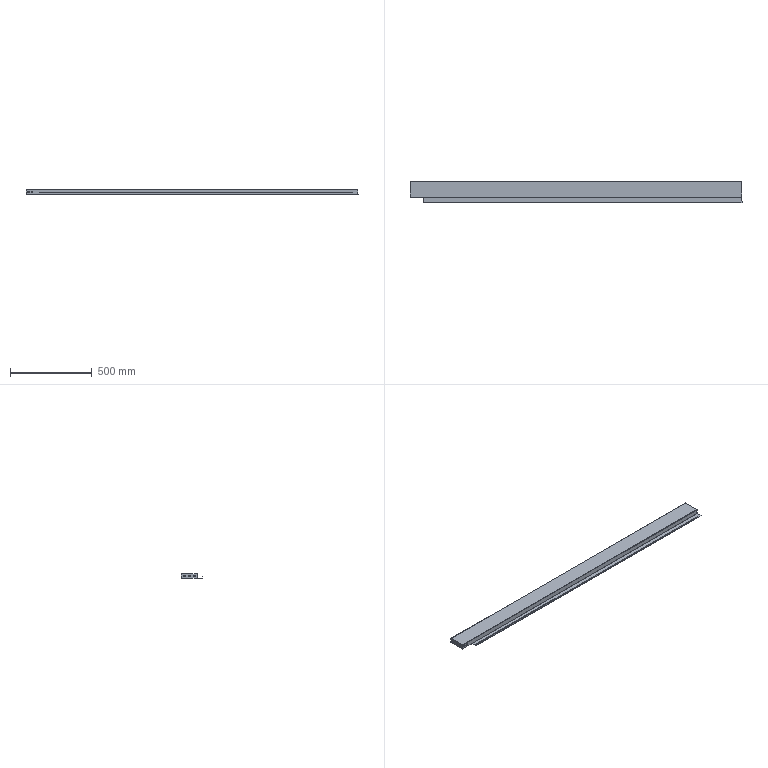Component | SolidWorks | UpperCrossbeam123-1 | 1 solid | 109 faces | volume 598632 mm3 | plane 64 | cylinder 45 | commonest cylinder face diameters 11 x33 3.4 x6 0.4 x6